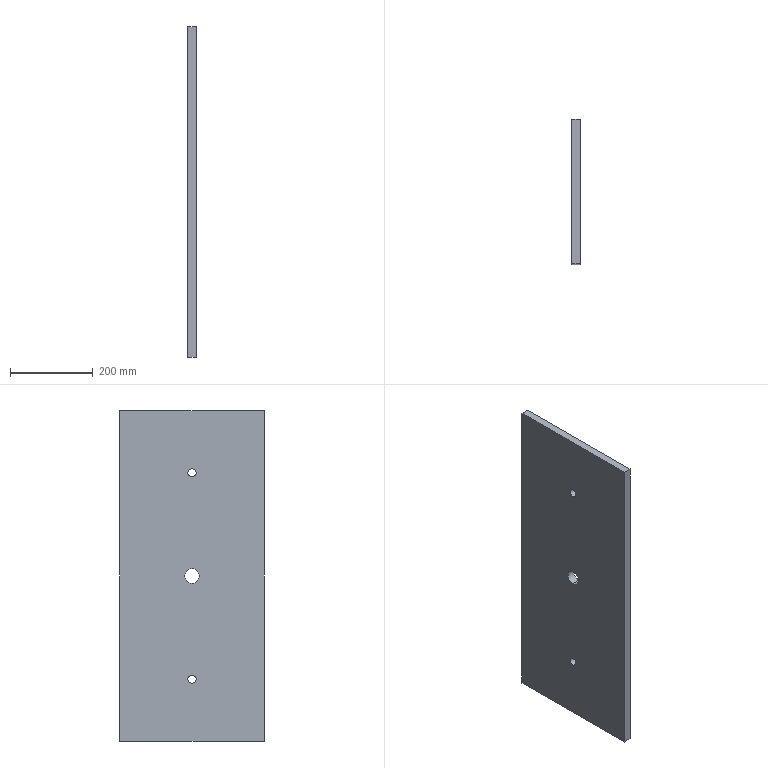Component | SolidWorks | ST60-08-1 | 1 solid | 12 faces | box 20 x 350 x 800 mm | volume 5568191 mm3 | cylinder 6 | plane 6 | commonest cylinder face diameters 20 x4 35 x2
build123d program:
from build123d import *

# Parameters (mm, degrees)
SKETCH1_W           = 800
SKETCH1_H           = 350
BOSS_EXTRUDE1_DEPTH = 20
SKETCH2_R           = 10
CUT_EXTRUDE1_DEPTH  = 1685.791
SKETCH3_R           = 17.5
CUT_EXTRUDE2_DEPTH  = 1685.791


with BuildPart() as part:
    # Sketch1 → Boss-Extrude1 (new body)
    with BuildSketch(Plane.XY):
        with Locations((-1124.489, 541.975)):
            Rectangle(SKETCH1_W, SKETCH1_H)
    extrude(amount=BOSS_EXTRUDE1_DEPTH)

    # Sketch2 → Cut-Extrude1 (cut, through all)
    with BuildSketch(Plane.XY.offset(20)):
        with Locations((-1374.489, 541.975)):
            Circle(SKETCH2_R)
        with Locations((-874.489, 541.975)):
            Circle(SKETCH2_R)
    extrude(amount=-CUT_EXTRUDE1_DEPTH, mode=Mode.SUBTRACT)

    # Sketch3 → Cut-Extrude2 (cut, through all)
    with BuildSketch(Plane.XY.offset(20)):
        with Locations((-1124.489, 541.975)):
            Circle(SKETCH3_R)
    extrude(amount=-CUT_EXTRUDE2_DEPTH, mode=Mode.SUBTRACT)


solid = part.part

# Placed as in the assembly
solid = solid.moved(Location((257.993, 68.479, -3025.889), (0, 90, 0)))
STEP:
#1=CARTESIAN_POINT('',(10.945,24.034,-75.547));
#2=VERTEX_POINT('',#1);
#3=CARTESIAN_POINT('',(10.945,24.034,-74.169));
#4=VERTEX_POINT('',#3);
#5=CARTESIAN_POINT('',(10.945,24.034,-74.858));
#6=DIRECTION('',(-1.,-0.,0.));
#7=DIRECTION('',(0.,0.,1.));
#8=AXIS2_PLACEMENT_3D('',#5,#6,#7);
#9=CIRCLE('',#8,0.689);
#10=EDGE_CURVE('',#2,#4,#9,.T.);
#11=ORIENTED_EDGE('',*,*,#10,.F.);
#12=CARTESIAN_POINT('',(10.157,24.034,-75.547));
#13=VERTEX_POINT('',#12);
#14=CARTESIAN_POINT('',(10.945,24.034,-75.547));
#15=DIRECTION('',(-1.,-0.,0.));
#16=VECTOR('',#15,39.37);
#17=LINE('',#14,#16);
#18=EDGE_CURVE('',#2,#13,#17,.T.);
#19=ORIENTED_EDGE('',*,*,#18,.T.);
#20=CARTESIAN_POINT('',(10.157,24.034,-74.169));
#21=VERTEX_POINT('',#20);
#22=CARTESIAN_POINT('',(10.157,24.034,-74.858));
#23=DIRECTION('',(-1.,-0.,0.));
#24=DIRECTION('',(0.,0.,1.));
#25=AXIS2_PLACEMENT_3D('',#22,#23,#24);
#26=CIRCLE('',#25,0.689);
#27=EDGE_CURVE('',#13,#21,#26,.T.);
#28=ORIENTED_EDGE('',*,*,#27,.T.);
#29=CARTESIAN_POINT('',(10.945,24.034,-74.169));
#30=DIRECTION('',(-1.,-0.,0.));
#31=VECTOR('',#30,39.37);
#32=LINE('',#29,#31);
#33=EDGE_CURVE('',#4,#21,#32,.T.);
#34=ORIENTED_EDGE('',*,*,#33,.F.);
#35=EDGE_LOOP('',(#11,#19,#28,#34));
#36=FACE_OUTER_BOUND('',#35,.T.);
#37=CARTESIAN_POINT('',(10.945,24.034,-74.858));
#38=DIRECTION('',(-1.,-0.,0.));
#39=DIRECTION('',(0.,0.,1.));
#40=AXIS2_PLACEMENT_3D('',#37,#38,#39);
#41=CYLINDRICAL_SURFACE('',#40,0.689);
#42=ADVANCED_FACE('',(#36),#41,.F.);
#43=CARTESIAN_POINT('',(10.945,24.034,-85.094));
#44=VERTEX_POINT('',#43);
#45=CARTESIAN_POINT('',(10.945,24.034,-84.307));
#46=VERTEX_POINT('',#45);
#47=CARTESIAN_POINT('',(10.945,24.034,-84.701));
#48=DIRECTION('',(-1.,-0.,0.));
#49=DIRECTION('',(0.,0.,1.));
#50=AXIS2_PLACEMENT_3D('',#47,#48,#49);
#51=CIRCLE('',#50,0.3937);
#52=EDGE_CURVE('',#44,#46,#51,.T.);
#53=ORIENTED_EDGE('',*,*,#52,.F.);
#54=CARTESIAN_POINT('',(10.157,24.034,-85.094));
#55=VERTEX_POINT('',#54);
#56=CARTESIAN_POINT('',(10.945,24.034,-85.094));
#57=DIRECTION('',(-1.,-0.,0.));
#58=VECTOR('',#57,39.37);
#59=LINE('',#56,#58);
#60=EDGE_CURVE('',#44,#55,#59,.T.);
#61=ORIENTED_EDGE('',*,*,#60,.T.);
#62=CARTESIAN_POINT('',(10.157,24.034,-84.307));
#63=VERTEX_POINT('',#62);
#64=CARTESIAN_POINT('',(10.157,24.034,-84.701));
#65=DIRECTION('',(-1.,-0.,0.));
#66=DIRECTION('',(0.,0.,1.));
#67=AXIS2_PLACEMENT_3D('',#64,#65,#66);
#68=CIRCLE('',#67,0.3937);
#69=EDGE_CURVE('',#55,#63,#68,.T.);
#70=ORIENTED_EDGE('',*,*,#69,.T.);
#71=CARTESIAN_POINT('',(10.945,24.034,-84.307));
#72=DIRECTION('',(-1.,-0.,0.));
#73=VECTOR('',#72,39.37);
#74=LINE('',#71,#73);
#75=EDGE_CURVE('',#46,#63,#74,.T.);
#76=ORIENTED_EDGE('',*,*,#75,.F.);
#77=EDGE_LOOP('',(#53,#61,#70,#76));
#78=FACE_OUTER_BOUND('',#77,.T.);
#79=CARTESIAN_POINT('',(10.945,24.034,-84.701));
#80=DIRECTION('',(-1.,-0.,0.));
#81=DIRECTION('',(0.,0.,1.));
#82=AXIS2_PLACEMENT_3D('',#79,#80,#81);
#83=CYLINDRICAL_SURFACE('',#82,0.3937);
#84=ADVANCED_FACE('',(#78),#83,.F.);
#85=CARTESIAN_POINT('',(10.945,24.034,-65.409));
#86=VERTEX_POINT('',#85);
#87=CARTESIAN_POINT('',(10.945,24.034,-64.622));
#88=VERTEX_POINT('',#87);
#89=CARTESIAN_POINT('',(10.945,24.034,-65.016));
#90=DIRECTION('',(-1.,-0.,0.));
#91=DIRECTION('',(0.,0.,1.));
#92=AXIS2_PLACEMENT_3D('',#89,#90,#91);
#93=CIRCLE('',#92,0.3937);
#94=EDGE_CURVE('',#86,#88,#93,.T.);
#95=ORIENTED_EDGE('',*,*,#94,.F.);
#96=CARTESIAN_POINT('',(10.157,24.034,-65.409));
#97=VERTEX_POINT('',#96);
#98=CARTESIAN_POINT('',(10.945,24.034,-65.409));
#99=DIRECTION('',(-1.,-0.,0.));
#100=VECTOR('',#99,39.37);
#101=LINE('',#98,#100);
#102=EDGE_CURVE('',#86,#97,#101,.T.);
#103=ORIENTED_EDGE('',*,*,#102,.T.);
#104=CARTESIAN_POINT('',(10.157,24.034,-64.622));
#105=VERTEX_POINT('',#104);
#106=CARTESIAN_POINT('',(10.157,24.034,-65.016));
#107=DIRECTION('',(-1.,-0.,0.));
#108=DIRECTION('',(0.,0.,1.));
#109=AXIS2_PLACEMENT_3D('',#106,#107,#108);
#110=CIRCLE('',#109,0.3937);
#111=EDGE_CURVE('',#97,#105,#110,.T.);
#112=ORIENTED_EDGE('',*,*,#111,.T.);
#113=CARTESIAN_POINT('',(10.945,24.034,-64.622));
#114=DIRECTION('',(-1.,-0.,0.));
#115=VECTOR('',#114,39.37);
#116=LINE('',#113,#115);
#117=EDGE_CURVE('',#88,#105,#116,.T.);
#118=ORIENTED_EDGE('',*,*,#117,.F.);
#119=EDGE_LOOP('',(#95,#103,#112,#118));
#120=FACE_OUTER_BOUND('',#119,.T.);
#121=CARTESIAN_POINT('',(10.945,24.034,-65.016));
#122=DIRECTION('',(-1.,-0.,0.));
#123=DIRECTION('',(0.,0.,1.));
#124=AXIS2_PLACEMENT_3D('',#121,#122,#123);
#125=CYLINDRICAL_SURFACE('',#124,0.3937);
#126=ADVANCED_FACE('',(#120),#125,.F.);
#127=CARTESIAN_POINT('',(10.945,30.923,-90.606));
#128=VERTEX_POINT('',#127);
#129=CARTESIAN_POINT('',(10.945,17.144,-90.606));
#130=VERTEX_POINT('',#129);
#131=CARTESIAN_POINT('',(10.945,30.923,-90.606));
#132=DIRECTION('',(0.,-1.,0.));
#133=VECTOR('',#132,39.37);
#134=LINE('',#131,#133);
#135=EDGE_CURVE('',#128,#130,#134,.T.);
#136=ORIENTED_EDGE('',*,*,#135,.T.);
#137=CARTESIAN_POINT('',(10.157,17.144,-90.606));
#138=VERTEX_POINT('',#137);
#139=CARTESIAN_POINT('',(10.157,17.144,-90.606));
#140=DIRECTION('',(1.,0.,-0.));
#141=VECTOR('',#140,39.37);
#142=LINE('',#139,#141);
#143=EDGE_CURVE('',#138,#130,#142,.T.);
#144=ORIENTED_EDGE('',*,*,#143,.F.);
#145=CARTESIAN_POINT('',(10.157,30.923,-90.606));
#146=VERTEX_POINT('',#145);
#147=CARTESIAN_POINT('',(10.157,30.923,-90.606));
#148=DIRECTION('',(0.,-1.,0.));
#149=VECTOR('',#148,39.37);
#150=LINE('',#147,#149);
#151=EDGE_CURVE('',#146,#138,#150,.T.);
#152=ORIENTED_EDGE('',*,*,#151,.F.);
#153=CARTESIAN_POINT('',(10.157,30.923,-90.606));
#154=DIRECTION('',(1.,0.,-0.));
#155=VECTOR('',#154,39.37);
#156=LINE('',#153,#155);
#157=EDGE_CURVE('',#146,#128,#156,.T.);
#158=ORIENTED_EDGE('',*,*,#157,.T.);
#159=EDGE_LOOP('',(#136,#144,#152,#158));
#160=FACE_OUTER_BOUND('',#159,.T.);
#161=CARTESIAN_POINT('',(10.157,30.923,-90.606));
#162=DIRECTION('',(0.,0.,1.));
#163=DIRECTION('',(-0.,1.,-0.));
#164=AXIS2_PLACEMENT_3D('',#161,#162,#163);
#165=PLANE('',#164);
#166=ADVANCED_FACE('',(#160),#165,.F.);
#167=CARTESIAN_POINT('',(10.945,17.144,-59.11));
#168=VERTEX_POINT('',#167);
#169=CARTESIAN_POINT('',(10.945,17.144,-90.606));
#170=DIRECTION('',(0.,-0.,1.));
#171=VECTOR('',#170,39.37);
#172=LINE('',#169,#171);
#173=EDGE_CURVE('',#130,#168,#172,.T.);
#174=ORIENTED_EDGE('',*,*,#173,.T.);
#175=CARTESIAN_POINT('',(10.157,17.144,-59.11));
#176=VERTEX_POINT('',#175);
#177=CARTESIAN_POINT('',(10.157,17.144,-59.11));
#178=DIRECTION('',(1.,0.,-0.));
#179=VECTOR('',#178,39.37);
#180=LINE('',#177,#179);
#181=EDGE_CURVE('',#176,#168,#180,.T.);
#182=ORIENTED_EDGE('',*,*,#181,.F.);
#183=CARTESIAN_POINT('',(10.157,17.144,-90.606));
#184=DIRECTION('',(0.,-0.,1.));
#185=VECTOR('',#184,39.37);
#186=LINE('',#183,#185);
#187=EDGE_CURVE('',#138,#176,#186,.T.);
#188=ORIENTED_EDGE('',*,*,#187,.F.);
#189=ORIENTED_EDGE('',*,*,#143,.T.);
#190=EDGE_LOOP('',(#174,#182,#188,#189));
#191=FACE_OUTER_BOUND('',#190,.T.);
#192=CARTESIAN_POINT('',(10.157,17.144,-90.606));
#193=DIRECTION('',(-0.,1.,0.));
#194=DIRECTION('',(-1.,-0.,0.));
#195=AXIS2_PLACEMENT_3D('',#192,#193,#194);
#196=PLANE('',#195);
#197=ADVANCED_FACE('',(#191),#196,.F.);
#198=CARTESIAN_POINT('',(10.945,30.923,-59.11));
#199=VERTEX_POINT('',#198);
#200=CARTESIAN_POINT('',(10.945,30.923,-59.11));
#201=DIRECTION('',(-0.,1.,0.));
#202=VECTOR('',#201,39.37);
#203=LINE('',#200,#202);
#204=EDGE_CURVE('',#168,#199,#203,.T.);
#205=ORIENTED_EDGE('',*,*,#204,.T.);
#206=CARTESIAN_POINT('',(10.157,30.923,-59.11));
#207=VERTEX_POINT('',#206);
#208=CARTESIAN_POINT('',(10.157,30.923,-59.11));
#209=DIRECTION('',(1.,0.,-0.));
#210=VECTOR('',#209,39.37);
#211=LINE('',#208,#210);
#212=EDGE_CURVE('',#207,#199,#211,.T.);
#213=ORIENTED_EDGE('',*,*,#212,.F.);
#214=CARTESIAN_POINT('',(10.157,30.923,-59.11));
#215=DIRECTION('',(-0.,1.,0.));
#216=VECTOR('',#215,39.37);
#217=LINE('',#214,#216);
#218=EDGE_CURVE('',#176,#207,#217,.T.);
#219=ORIENTED_EDGE('',*,*,#218,.F.);
#220=ORIENTED_EDGE('',*,*,#181,.T.);
#221=EDGE_LOOP('',(#205,#213,#219,#220));
#222=FACE_OUTER_BOUND('',#221,.T.);
#223=CARTESIAN_POINT('',(10.157,30.923,-59.11));
#224=DIRECTION('',(-0.,0.,-1.));
#225=DIRECTION('',(-1.,-0.,0.));
#226=AXIS2_PLACEMENT_3D('',#223,#224,#225);
#227=PLANE('',#226);
#228=ADVANCED_FACE('',(#222),#227,.F.);
#229=CARTESIAN_POINT('',(10.945,30.923,-90.606));
#230=DIRECTION('',(-0.,0.,-1.));
#231=VECTOR('',#230,39.37);
#232=LINE('',#229,#231);
#233=EDGE_CURVE('',#199,#128,#232,.T.);
#234=ORIENTED_EDGE('',*,*,#233,.T.);
#235=ORIENTED_EDGE('',*,*,#157,.F.);
#236=CARTESIAN_POINT('',(10.157,30.923,-90.606));
#237=DIRECTION('',(-0.,0.,-1.));
#238=VECTOR('',#237,39.37);
#239=LINE('',#236,#238);
#240=EDGE_CURVE('',#207,#146,#239,.T.);
#241=ORIENTED_EDGE('',*,*,#240,.F.);
#242=ORIENTED_EDGE('',*,*,#212,.T.);
#243=EDGE_LOOP('',(#234,#235,#241,#242));
#244=FACE_OUTER_BOUND('',#243,.T.);
#245=CARTESIAN_POINT('',(10.157,30.923,-90.606));
#246=DIRECTION('',(0.,-1.,-0.));
#247=DIRECTION('',(1.,0.,-0.));
#248=AXIS2_PLACEMENT_3D('',#245,#246,#247);
#249=PLANE('',#248);
#250=ADVANCED_FACE('',(#244),#249,.F.);
#251=CARTESIAN_POINT('',(10.157,24.034,-74.858));
#252=DIRECTION('',(-1.,-0.,0.));
#253=DIRECTION('',(0.,0.,1.));
#254=AXIS2_PLACEMENT_3D('',#251,#252,#253);
#255=CIRCLE('',#254,0.689);
#256=EDGE_CURVE('',#21,#13,#255,.T.);
#257=ORIENTED_EDGE('',*,*,#256,.F.);
#258=ORIENTED_EDGE('',*,*,#27,.F.);
#259=EDGE_LOOP('',(#257,#258));
#260=FACE_BOUND('',#259,.T.);
#261=CARTESIAN_POINT('',(10.157,24.034,-84.701));
#262=DIRECTION('',(-1.,-0.,0.));
#263=DIRECTION('',(0.,0.,1.));
#264=AXIS2_PLACEMENT_3D('',#261,#262,#263);
#265=CIRCLE('',#264,0.3937);
#266=EDGE_CURVE('',#63,#55,#265,.T.);
#267=ORIENTED_EDGE('',*,*,#266,.F.);
#268=ORIENTED_EDGE('',*,*,#69,.F.);
#269=EDGE_LOOP('',(#267,#268));
#270=FACE_BOUND('',#269,.T.);
#271=CARTESIAN_POINT('',(10.157,24.034,-65.016));
#272=DIRECTION('',(-1.,-0.,0.));
#273=DIRECTION('',(0.,0.,1.));
#274=AXIS2_PLACEMENT_3D('',#271,#272,#273);
#275=CIRCLE('',#274,0.3937);
#276=EDGE_CURVE('',#105,#97,#275,.T.);
#277=ORIENTED_EDGE('',*,*,#276,.F.);
#278=ORIENTED_EDGE('',*,*,#111,.F.);
#279=EDGE_LOOP('',(#277,#278));
#280=FACE_BOUND('',#279,.T.);
#281=ORIENTED_EDGE('',*,*,#151,.T.);
#282=ORIENTED_EDGE('',*,*,#187,.T.);
#283=ORIENTED_EDGE('',*,*,#218,.T.);
#284=ORIENTED_EDGE('',*,*,#240,.T.);
#285=EDGE_LOOP('',(#281,#282,#283,#284));
#286=FACE_OUTER_BOUND('',#285,.T.);
#287=CARTESIAN_POINT('',(10.157,2.696,-30.587));
#288=DIRECTION('',(-1.,-0.,0.));
#289=DIRECTION('',(0.,-0.,1.));
#290=AXIS2_PLACEMENT_3D('',#287,#288,#289);
#291=PLANE('',#290);
#292=ADVANCED_FACE('',(#260,#270,#280,#286),#291,.T.);
#293=CARTESIAN_POINT('',(10.945,24.034,-74.858));
#294=DIRECTION('',(-1.,-0.,0.));
#295=DIRECTION('',(0.,0.,1.));
#296=AXIS2_PLACEMENT_3D('',#293,#294,#295);
#297=CIRCLE('',#296,0.689);
#298=EDGE_CURVE('',#4,#2,#297,.T.);
#299=ORIENTED_EDGE('',*,*,#298,.T.);
#300=ORIENTED_EDGE('',*,*,#10,.T.);
#301=EDGE_LOOP('',(#299,#300));
#302=FACE_BOUND('',#301,.T.);
#303=CARTESIAN_POINT('',(10.945,24.034,-84.701));
#304=DIRECTION('',(-1.,-0.,0.));
#305=DIRECTION('',(0.,0.,1.));
#306=AXIS2_PLACEMENT_3D('',#303,#304,#305);
#307=CIRCLE('',#306,0.3937);
#308=EDGE_CURVE('',#46,#44,#307,.T.);
#309=ORIENTED_EDGE('',*,*,#308,.T.);
#310=ORIENTED_EDGE('',*,*,#52,.T.);
#311=EDGE_LOOP('',(#309,#310));
#312=FACE_BOUND('',#311,.T.);
#313=CARTESIAN_POINT('',(10.945,24.034,-65.016));
#314=DIRECTION('',(-1.,-0.,0.));
#315=DIRECTION('',(0.,0.,1.));
#316=AXIS2_PLACEMENT_3D('',#313,#314,#315);
#317=CIRCLE('',#316,0.3937);
#318=EDGE_CURVE('',#88,#86,#317,.T.);
#319=ORIENTED_EDGE('',*,*,#318,.T.);
#320=ORIENTED_EDGE('',*,*,#94,.T.);
#321=EDGE_LOOP('',(#319,#320));
#322=FACE_BOUND('',#321,.T.);
#323=ORIENTED_EDGE('',*,*,#135,.F.);
#324=ORIENTED_EDGE('',*,*,#233,.F.);
#325=ORIENTED_EDGE('',*,*,#204,.F.);
#326=ORIENTED_EDGE('',*,*,#173,.F.);
#327=EDGE_LOOP('',(#323,#324,#325,#326));
#328=FACE_OUTER_BOUND('',#327,.T.);
#329=CARTESIAN_POINT('',(10.945,2.696,-30.587));
#330=DIRECTION('',(-1.,-0.,0.));
#331=DIRECTION('',(0.,-0.,1.));
#332=AXIS2_PLACEMENT_3D('',#329,#330,#331);
#333=PLANE('',#332);
#334=ADVANCED_FACE('',(#302,#312,#322,#328),#333,.F.);
#335=ORIENTED_EDGE('',*,*,#102,.F.);
#336=ORIENTED_EDGE('',*,*,#318,.F.);
#337=ORIENTED_EDGE('',*,*,#117,.T.);
#338=ORIENTED_EDGE('',*,*,#276,.T.);
#339=EDGE_LOOP('',(#335,#336,#337,#338));
#340=FACE_OUTER_BOUND('',#339,.T.);
#341=CARTESIAN_POINT('',(10.945,24.034,-65.016));
#342=DIRECTION('',(-1.,-0.,0.));
#343=DIRECTION('',(0.,0.,1.));
#344=AXIS2_PLACEMENT_3D('',#341,#342,#343);
#345=CYLINDRICAL_SURFACE('',#344,0.3937);
#346=ADVANCED_FACE('',(#340),#345,.F.);
#347=ORIENTED_EDGE('',*,*,#60,.F.);
#348=ORIENTED_EDGE('',*,*,#308,.F.);
#349=ORIENTED_EDGE('',*,*,#75,.T.);
#350=ORIENTED_EDGE('',*,*,#266,.T.);
#351=EDGE_LOOP('',(#347,#348,#349,#350));
#352=FACE_OUTER_BOUND('',#351,.T.);
#353=CARTESIAN_POINT('',(10.945,24.034,-84.701));
#354=DIRECTION('',(-1.,-0.,0.));
#355=DIRECTION('',(0.,0.,1.));
#356=AXIS2_PLACEMENT_3D('',#353,#354,#355);
#357=CYLINDRICAL_SURFACE('',#356,0.3937);
#358=ADVANCED_FACE('',(#352),#357,.F.);
#359=ORIENTED_EDGE('',*,*,#18,.F.);
#360=ORIENTED_EDGE('',*,*,#298,.F.);
#361=ORIENTED_EDGE('',*,*,#33,.T.);
#362=ORIENTED_EDGE('',*,*,#256,.T.);
#363=EDGE_LOOP('',(#359,#360,#361,#362));
#364=FACE_OUTER_BOUND('',#363,.T.);
#365=CARTESIAN_POINT('',(10.945,24.034,-74.858));
#366=DIRECTION('',(-1.,-0.,0.));
#367=DIRECTION('',(0.,0.,1.));
#368=AXIS2_PLACEMENT_3D('',#365,#366,#367);
#369=CYLINDRICAL_SURFACE('',#368,0.689);
#370=ADVANCED_FACE('',(#364),#369,.F.);
#371=CLOSED_SHELL('',(#42,#84,#126,#166,#197,#228,#250,#292,#334,#346,#358,#370));
#372=MANIFOLD_SOLID_BREP('',#371);
#373=CARTESIAN_POINT('',(0.,0.,0.));
#374=DIRECTION('',(0.,0.,1.));
#375=DIRECTION('',(1.,0.,0.));
#376=AXIS2_PLACEMENT_3D('',#373,#374,#375);
#377=(LENGTH_UNIT()NAMED_UNIT(*)SI_UNIT($,.METRE.));
#378=LENGTH_MEASURE_WITH_UNIT(LENGTH_MEASURE(0.0254),#377);
#379=DIMENSIONAL_EXPONENTS(1.,0.,0.,0.,0.,0.,0.);
#380=(CONVERSION_BASED_UNIT('',#378)LENGTH_UNIT()NAMED_UNIT(#379));
#381=UNCERTAINTY_MEASURE_WITH_UNIT(LENGTH_MEASURE(0.00001),#380,'','');
#382=(NAMED_UNIT(*)PLANE_ANGLE_UNIT()SI_UNIT($,.RADIAN.));
#383=(NAMED_UNIT(*)SI_UNIT($,.STERADIAN.)SOLID_ANGLE_UNIT());
#384=(GEOMETRIC_REPRESENTATION_CONTEXT(3)GLOBAL_UNCERTAINTY_ASSIGNED_CONTEXT((#381))GLOBAL_UNIT_ASSIGNED_CONTEXT((#380,#382,#383))REPRESENTATION_CONTEXT('',''));
#385=ADVANCED_BREP_SHAPE_REPRESENTATION('',(#372,#376),#384);
#386=COLOUR_RGB('',0.7922,0.8196,0.9333);
#387=FILL_AREA_STYLE_COLOUR('',#386);
#388=FILL_AREA_STYLE('',(#387));
#389=SURFACE_STYLE_FILL_AREA(#388);
#390=SURFACE_SIDE_STYLE('',(#389));
#391=SURFACE_STYLE_USAGE(.BOTH.,#390);
#392=PRESENTATION_STYLE_ASSIGNMENT((#391));
#393=STYLED_ITEM('',(#392),#372);
#394=(LENGTH_UNIT()NAMED_UNIT(*)SI_UNIT($,.METRE.));
#395=LENGTH_MEASURE_WITH_UNIT(LENGTH_MEASURE(0.0254),#394);
#396=DIMENSIONAL_EXPONENTS(1.,0.,0.,0.,0.,0.,0.);
#397=(CONVERSION_BASED_UNIT('',#395)LENGTH_UNIT()NAMED_UNIT(#396));
#398=UNCERTAINTY_MEASURE_WITH_UNIT(LENGTH_MEASURE(0.00001),#397,'','');
#399=(NAMED_UNIT(*)PLANE_ANGLE_UNIT()SI_UNIT($,.RADIAN.));
#400=(NAMED_UNIT(*)SI_UNIT($,.STERADIAN.)SOLID_ANGLE_UNIT());
#401=(GEOMETRIC_REPRESENTATION_CONTEXT(3)GLOBAL_UNCERTAINTY_ASSIGNED_CONTEXT((#398))GLOBAL_UNIT_ASSIGNED_CONTEXT((#397,#399,#400))REPRESENTATION_CONTEXT('',''));
#402=MECHANICAL_DESIGN_GEOMETRIC_PRESENTATION_REPRESENTATION('',(#393),#401);
#403=PRESENTATION_LAYER_ASSIGNMENT('','',(#393));